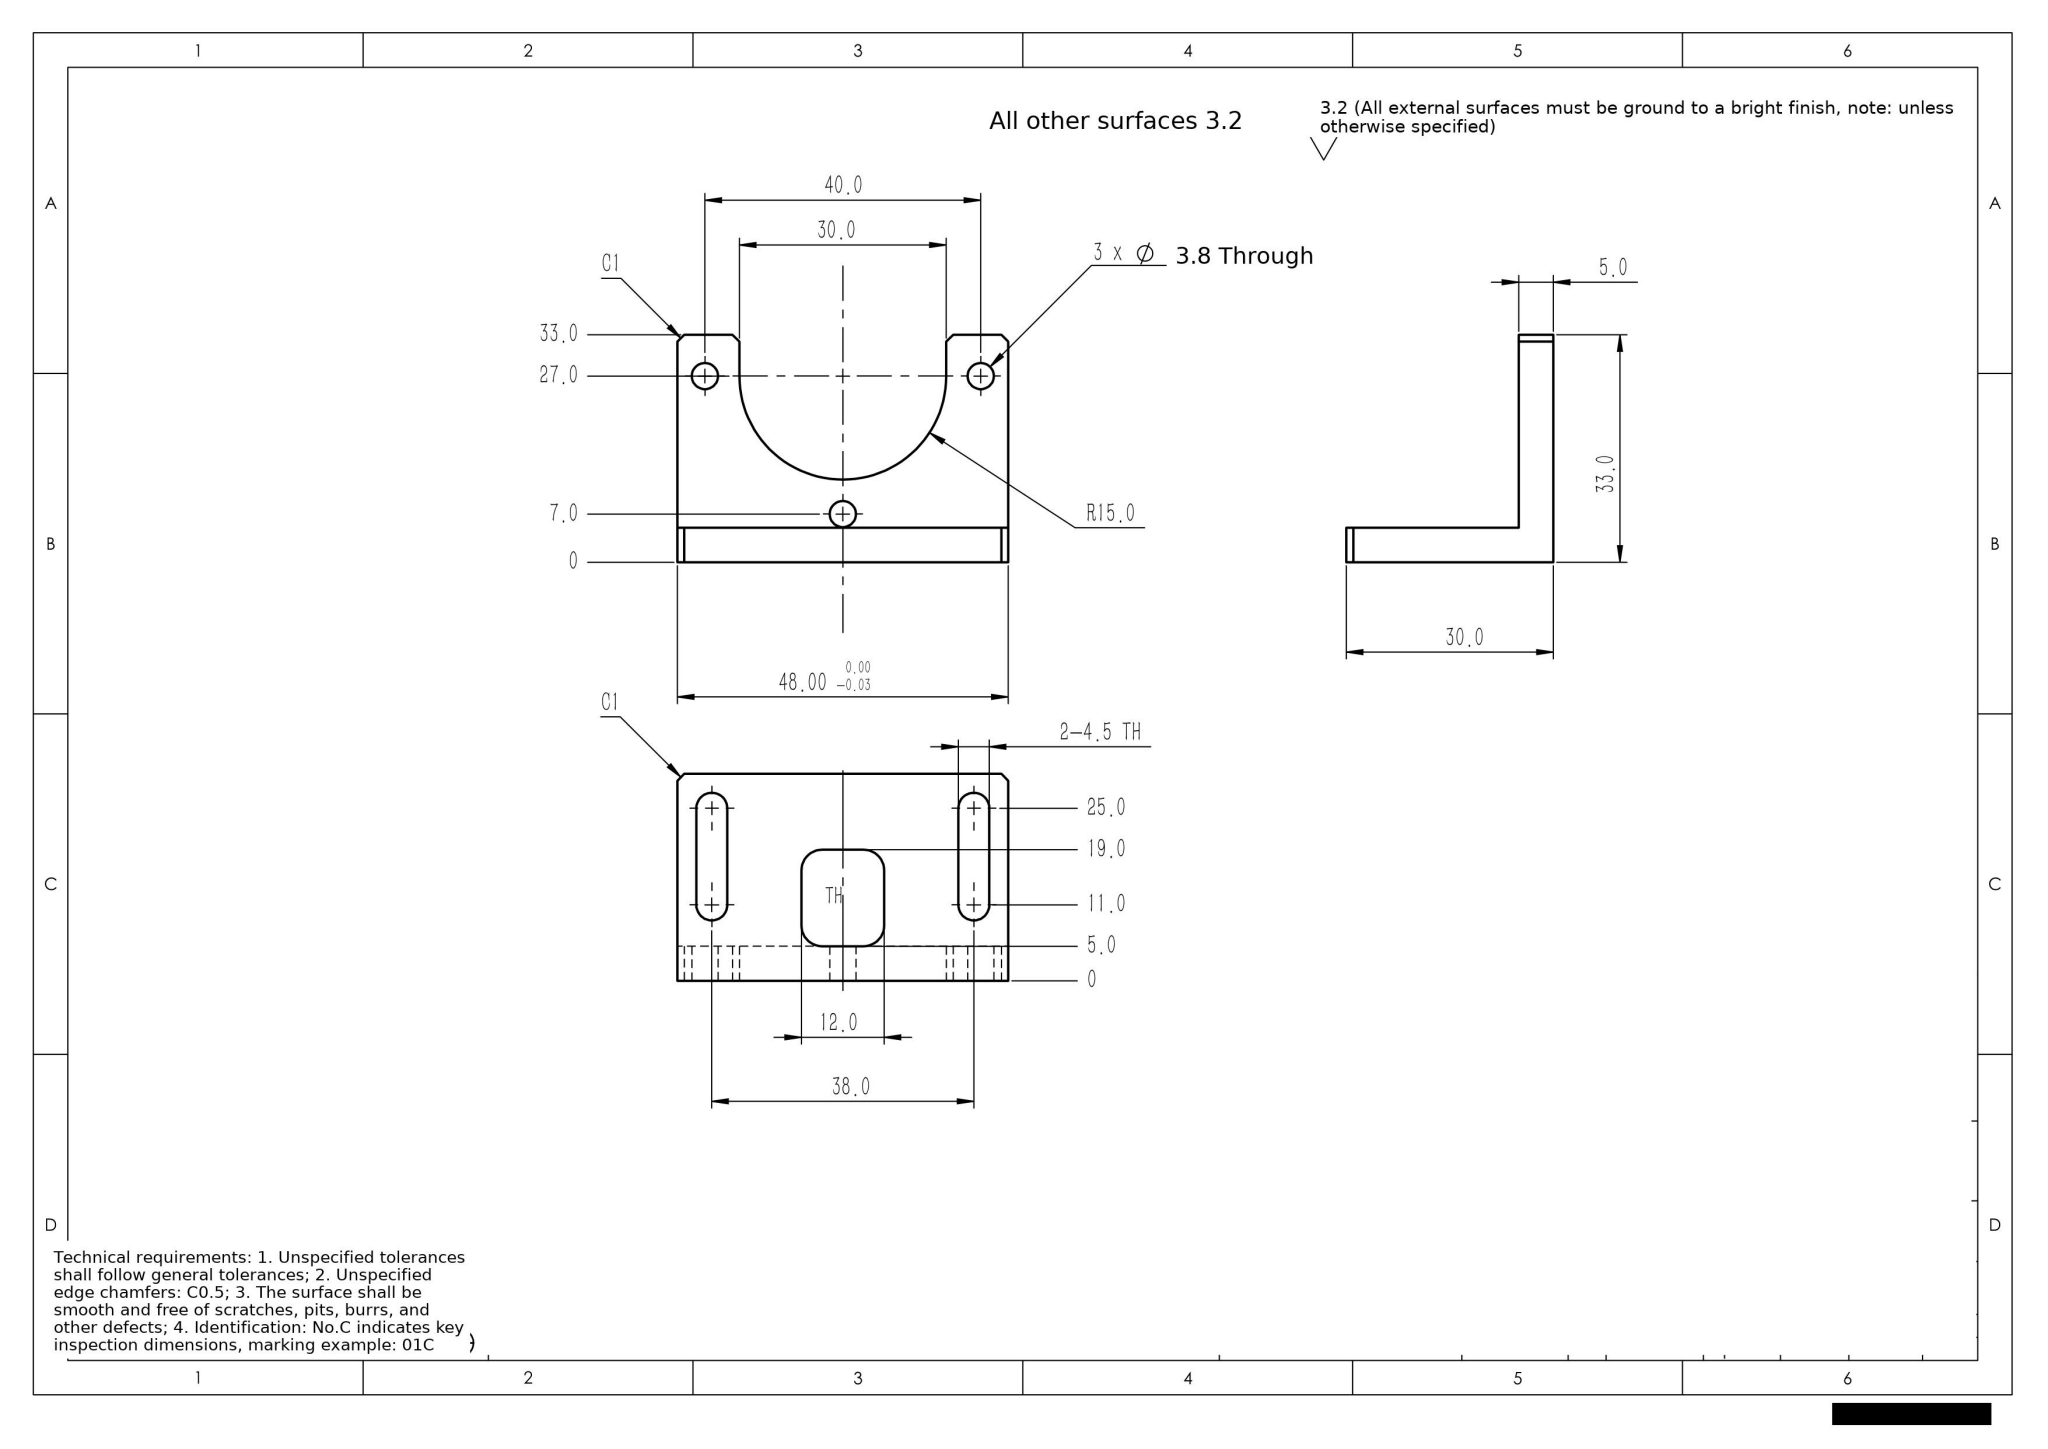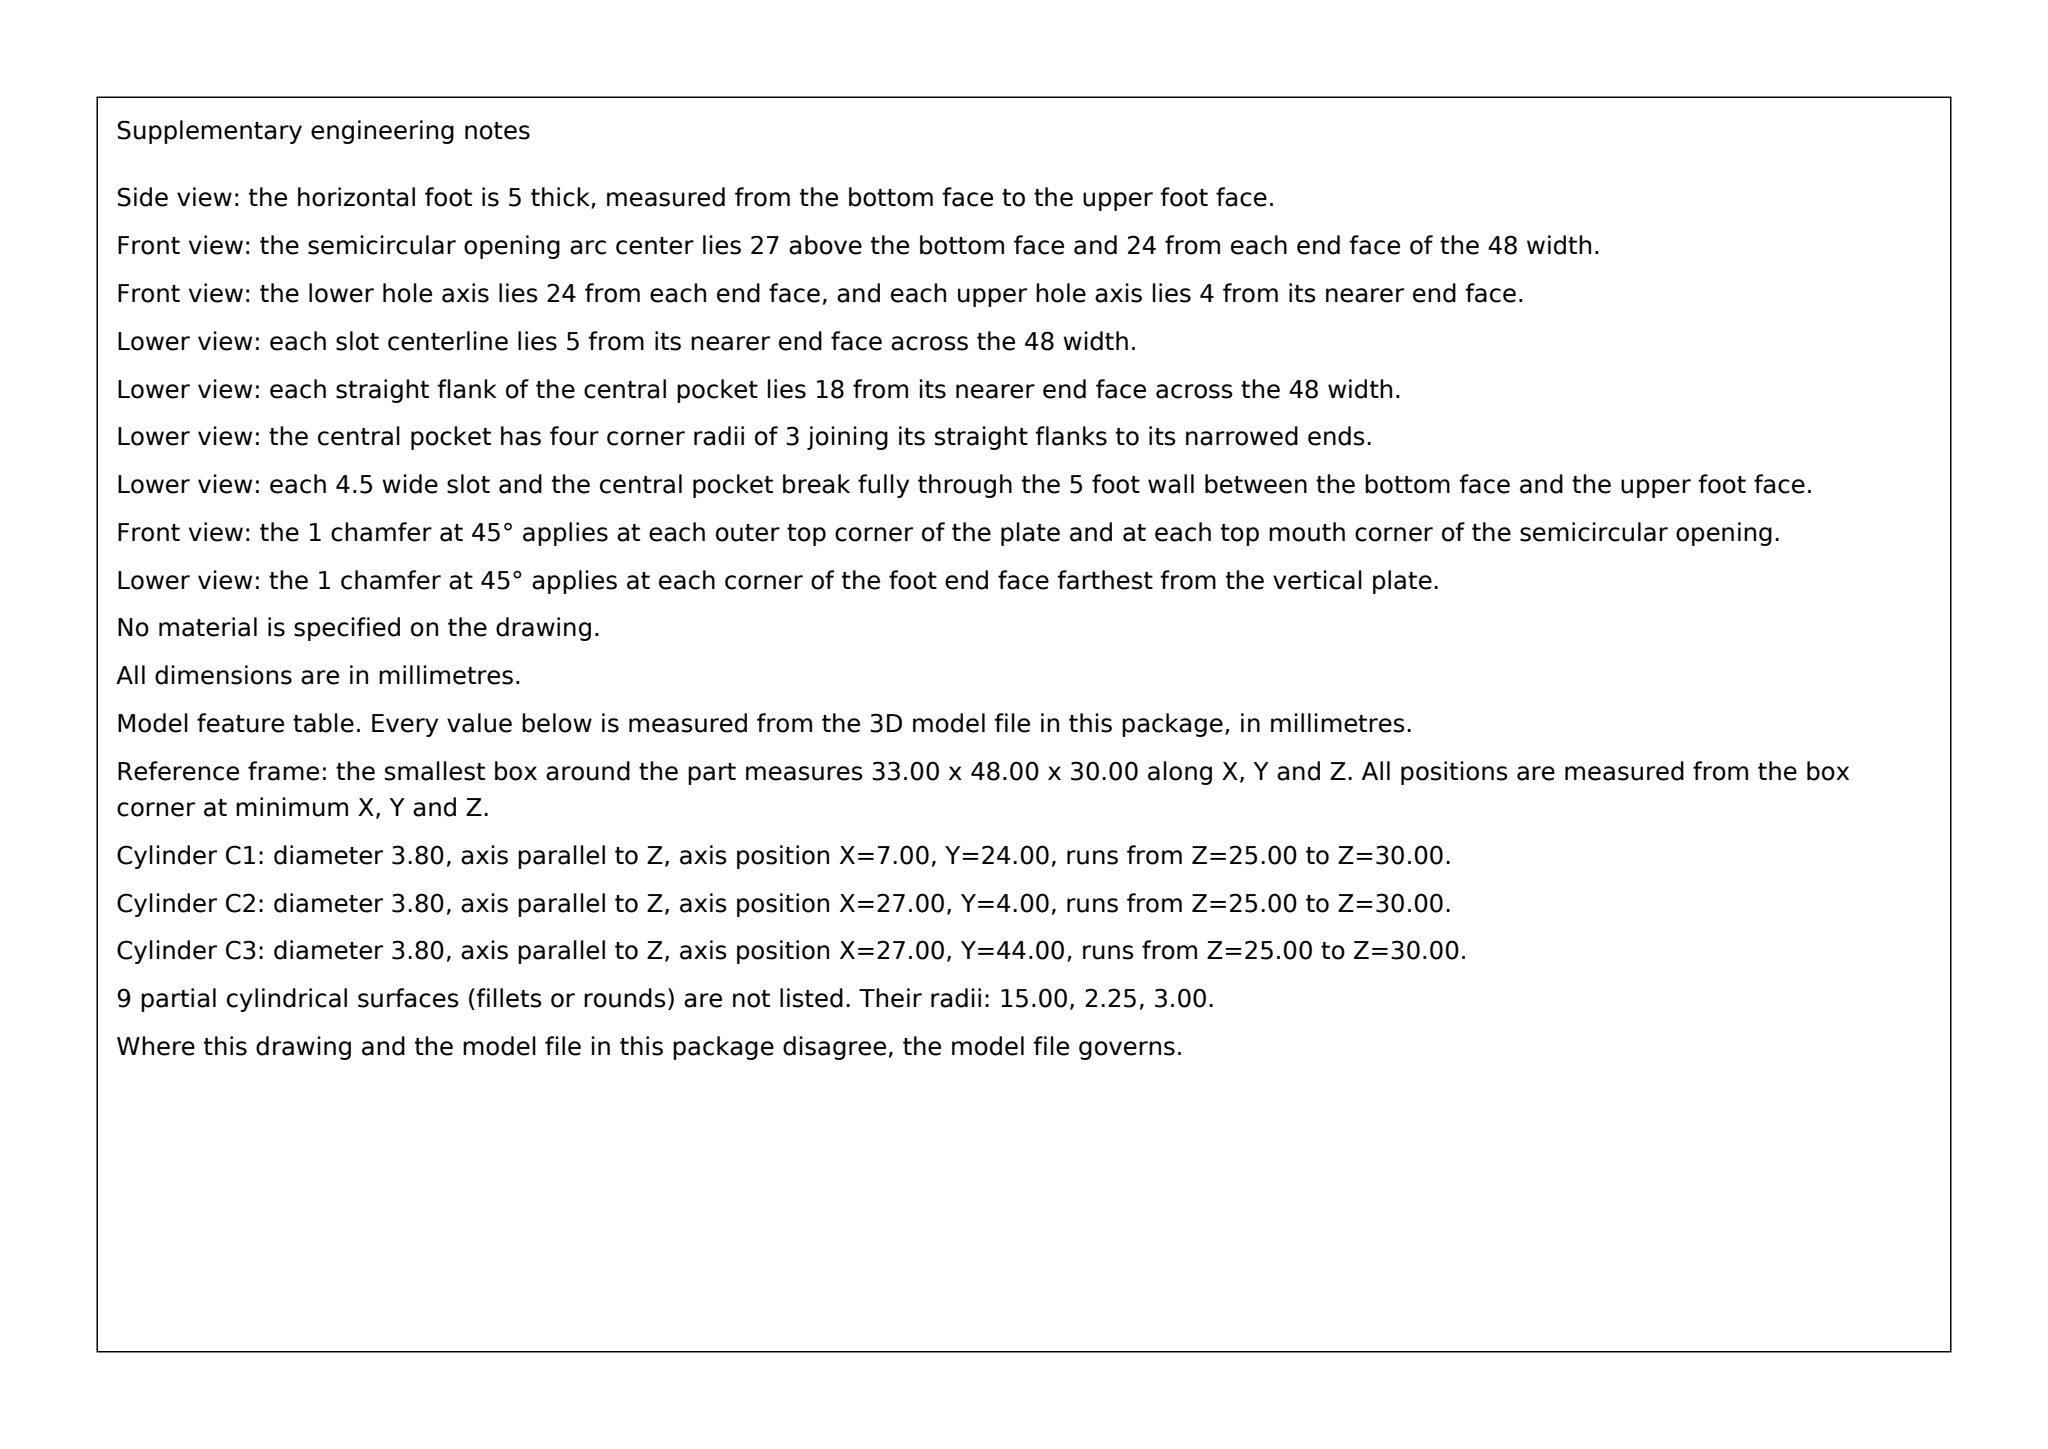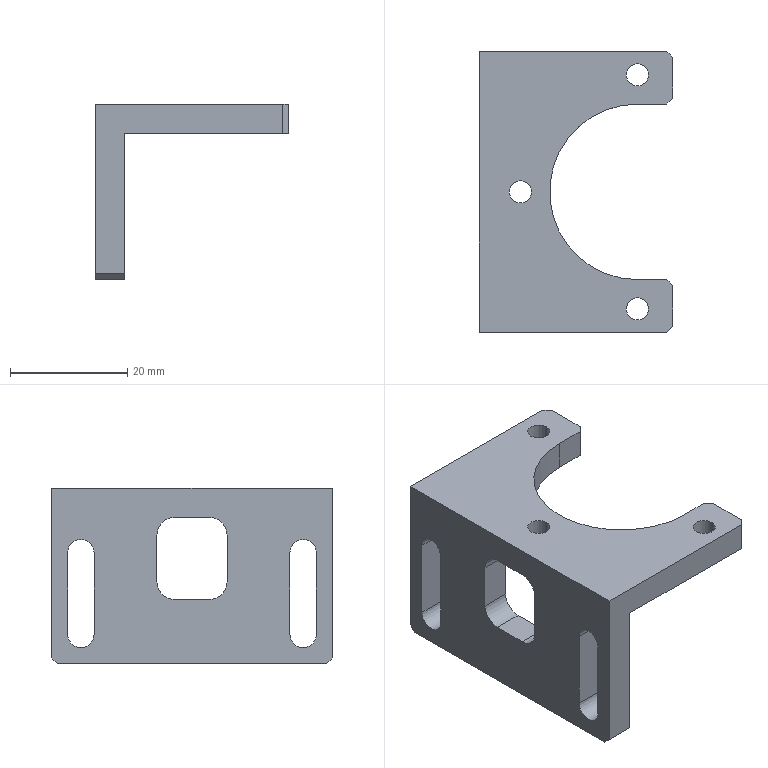Part | SolidWorks | mm | 1 solid | 41 faces | box 33 x 48 x 30 mm | volume 9477 mm3 | plane 24 | cylinder 17 | commonest cylinder face diameters 3.8 x6 4.5 x6 6 x4 30 x1
Drawing notes:
(3) 2X C1 AT ENDS OF 30.0 OPENING, TOP FACE (4X C1 TOP TOTAL) | from the solid: Inclined 45 deg planes 1x1x5 at bbox_from [32,8,25] & [32,39,25] (notch corners); plus [32,0,25] & [32,47,25] outer corners
(2) BASE PLATE THK 5.0; VERT PLATE THK 5.0 | from the solid: Planes x=0 (y0-48,z0-30) and x=5 (y0-48,z0-25) -> 5.0 base thk; planes z=25 and z=30 -> 5.0 vert plate thk
(1) 4X R3.0 POCKET CORNERS, POCKET 12.0 x 14.0 THRU | from the solid: Four 90 deg arcs dia 6.0 axis x at y=21/27, z=14/22, x 0-5; pocket walls y=18 & y=30, end z=11, open to z=25
2X Ø4.5 SLOT, 14.0 LG, THRU 5.0 BASE PLATE | from the solid: 180 deg arcs dia 4.5 axis x at (y43,z19),(y43,z5),(y5,z19),(y5,z5), x 0-5; side walls y=2.8/7.2 and y=40.8/45.2, z 5-19
POCKET 12.0 WIDE x 14.0 LG, R3.0 CORNERS, THRU 5.0 BASE | from the solid: Pocket faces y=18/y=30 (12.0 wide), z=11 end to z=25, x 0-5 through, 4X R3.0 corner arcs
build123d program:
from build123d import *

# Parameters (mm, degrees)
BOSS_EXTRUDE1_DEPTH        = 24
CUT_EXTRUDE1_DEPTH         = 51.646
CUT_EXTRUDE1_DEPTH_BACK    = 51.646
CUT_EXTRUDE2_DEPTH         = 51.646
F_3_8_3_8_DIAMETER_HOLE1_D = 3.8
SKETCH9_W                  = 14
SKETCH9_H                  = 12
CUT_EXTRUDE3_DEPTH         = 51.646
FILLET1_R                  = 3
CHAMFER1_SIZE              = 1


with BuildPart() as part:
    # Sketch1 → Boss-Extrude1 (new, symmetric)
    with BuildSketch(Plane(origin=(0, 0, 0), x_dir=(1, 0, 0), z_dir=(0, 1, 0))):
        Polygon((0, 0), (33, 0), (33, 5), (5, 5), (5, 30), (0, 30), align=None)
    extrude(amount=BOSS_EXTRUDE1_DEPTH, both=True)

    # Sketch2 → Cut-Extrude1 (cut, two sides: drawn at the far end of the back side and taken through both)
    with BuildSketch(Plane.ZY.offset(-CUT_EXTRUDE1_DEPTH_BACK)):
        with BuildLine():
            Line((-11, 16.75), (-25, 16.75))
            ThreePointArc((-25, 16.75), (-27.25, 19), (-25, 21.25))
            Line((-25, 21.25), (-11, 21.25))
            ThreePointArc((-11, 21.25), (-8.75, 19), (-11, 16.75))
        make_face()
        with BuildLine():
            Line((-11, -21.25), (-25, -21.25))
            ThreePointArc((-25, -21.25), (-27.25, -19), (-25, -16.75))
            Line((-25, -16.75), (-11, -16.75))
            ThreePointArc((-11, -16.75), (-8.75, -19), (-11, -21.25))
        make_face()
    extrude(amount=CUT_EXTRUDE1_DEPTH + CUT_EXTRUDE1_DEPTH_BACK, mode=Mode.SUBTRACT)

    # Sketch3 → Cut-Extrude2 (cut, through all)
    with BuildSketch(Plane.XY):
        with BuildLine():
            Line((42, -15), (27, -15))
            ThreePointArc((27, -15), (12, 0), (27, 15))
            Line((27, 15), (42, 15))
            ThreePointArc((42, 15), (57, 0), (42, -15))
        make_face()
    extrude(amount=-CUT_EXTRUDE2_DEPTH, mode=Mode.SUBTRACT)

    # 3.8 _3.8_ Diameter Hole1 (through all)
    with Locations(Plane.XY):
        with Locations((27, 20), (7, 0), (27, -20)):
            Hole(F_3_8_3_8_DIAMETER_HOLE1_D / 2)

    # Sketch9 → Cut-Extrude3 (cut, through all)
    with BuildSketch(Plane.ZY):
        with Locations((-12, 0)):
            Rectangle(SKETCH9_W, SKETCH9_H)
    extrude(amount=-CUT_EXTRUDE3_DEPTH, mode=Mode.SUBTRACT)

    # Fillet1
    fillet1_edges = [part.edges().sort_by_distance(p)[0] for p in [
        (2.5, -6, -5),
        (2.5, -6, -19),
        (2.5, 6, -19),
        (2.5, 6, -5),
    ]]
    fillet(fillet1_edges, radius=FILLET1_R)

    # Chamfer1
    chamfer1_edges = [part.edges().sort_by_distance(p)[0] for p in [
        (33, 24, -2.5),
        (2.5, 24, -30),
        (2.5, -24, -30),
        (33, -15, -2.5),
        (33, 15, -2.5),
        (33, -24, -2.5),
    ]]
    chamfer(chamfer1_edges, length=CHAMFER1_SIZE)


solid = part.part